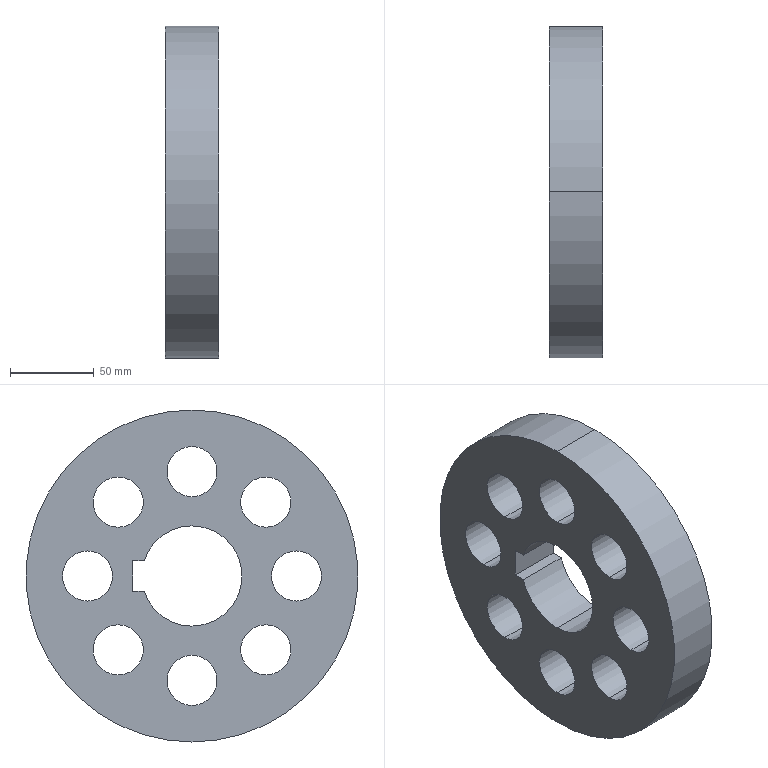Component | SolidWorks | SynchronousDrivePulley-1 | 1 solid | 26 faces | box 32 x 198.68 x 198.68 mm | volume 717277 mm3 | cylinder 21 | plane 5 | commonest cylinder face diameters 30 x16 60 x3 198.68 x2
build123d program:
from build123d import *

# Parameters (mm, degrees)
SKETCH1_R           = 99.34
SKETCH1_R_2         = 15
BOSS_EXTRUDE1_DEPTH = 16


with BuildPart() as part:
    # Sketch1 → Boss-Extrude1 (new, symmetric)
    with BuildSketch(Plane(origin=(0, 0, 0), x_dir=(0, 0, -1), z_dir=(1, 0, 0))):
        Circle(SKETCH1_R)
        with Locations((0, 62.5)):
            Circle(SKETCH1_R_2, mode=Mode.SUBTRACT)
        with Locations((44.194, 44.194)):
            Circle(SKETCH1_R_2, mode=Mode.SUBTRACT)
        with Locations((62.5, 0)):
            Circle(SKETCH1_R_2, mode=Mode.SUBTRACT)
        with Locations((44.194, -44.194)):
            Circle(SKETCH1_R_2, mode=Mode.SUBTRACT)
        with Locations((0, -62.5)):
            Circle(SKETCH1_R_2, mode=Mode.SUBTRACT)
        with Locations((-44.194, -44.194)):
            Circle(SKETCH1_R_2, mode=Mode.SUBTRACT)
        with Locations((-62.5, 0)):
            Circle(SKETCH1_R_2, mode=Mode.SUBTRACT)
        with Locations((-44.194, 44.194)):
            Circle(SKETCH1_R_2, mode=Mode.SUBTRACT)
        with BuildLine():
            Line((-9, 35.4), (9, 35.4))
            Line((9, 35.4), (9, 28.618))
            ThreePointArc((9, 28.618), (0, -30), (-9, 28.618))
            Line((-9, 28.618), (-9, 35.4))
        make_face(mode=Mode.SUBTRACT)
    extrude(amount=BOSS_EXTRUDE1_DEPTH, both=True)


solid = part.part

# Placed as in the assembly
solid = solid.moved(Location((518.553, 34.532, 0), (0, 0, 0)))
STEP:
#1=CARTESIAN_POINT('',(21.045,3.099,2.33));
#2=VERTEX_POINT('',#1);
#3=CARTESIAN_POINT('',(21.045,3.099,1.149));
#4=VERTEX_POINT('',#3);
#5=CARTESIAN_POINT('',(21.045,3.099,1.74));
#6=DIRECTION('',(1.,0.,0.));
#7=DIRECTION('',(0.,0.,-1.));
#8=AXIS2_PLACEMENT_3D('',#5,#6,#7);
#9=CIRCLE('',#8,0.5906);
#10=EDGE_CURVE('',#2,#4,#9,.T.);
#11=ORIENTED_EDGE('',*,*,#10,.T.);
#12=CARTESIAN_POINT('',(19.786,3.099,1.149));
#13=VERTEX_POINT('',#12);
#14=CARTESIAN_POINT('',(21.045,3.099,1.149));
#15=DIRECTION('',(-1.,0.,0.));
#16=VECTOR('',#15,39.37);
#17=LINE('',#14,#16);
#18=EDGE_CURVE('',#4,#13,#17,.T.);
#19=ORIENTED_EDGE('',*,*,#18,.T.);
#20=CARTESIAN_POINT('',(19.786,3.099,2.33));
#21=VERTEX_POINT('',#20);
#22=CARTESIAN_POINT('',(19.786,3.099,1.74));
#23=DIRECTION('',(1.,0.,0.));
#24=DIRECTION('',(0.,0.,-1.));
#25=AXIS2_PLACEMENT_3D('',#22,#23,#24);
#26=CIRCLE('',#25,0.5906);
#27=EDGE_CURVE('',#21,#13,#26,.T.);
#28=ORIENTED_EDGE('',*,*,#27,.F.);
#29=CARTESIAN_POINT('',(21.045,3.099,2.33));
#30=DIRECTION('',(-1.,0.,0.));
#31=VECTOR('',#30,39.37);
#32=LINE('',#29,#31);
#33=EDGE_CURVE('',#2,#21,#32,.T.);
#34=ORIENTED_EDGE('',*,*,#33,.F.);
#35=EDGE_LOOP('',(#11,#19,#28,#34));
#36=FACE_OUTER_BOUND('',#35,.T.);
#37=CARTESIAN_POINT('',(21.045,3.099,1.74));
#38=DIRECTION('',(-1.,0.,0.));
#39=DIRECTION('',(0.,0.,1.));
#40=AXIS2_PLACEMENT_3D('',#37,#38,#39);
#41=CYLINDRICAL_SURFACE('',#40,0.5906);
#42=ADVANCED_FACE('',(#36),#41,.F.);
#43=CARTESIAN_POINT('',(21.045,1.36,3.051));
#44=VERTEX_POINT('',#43);
#45=CARTESIAN_POINT('',(21.045,1.36,1.87));
#46=VERTEX_POINT('',#45);
#47=CARTESIAN_POINT('',(21.045,1.36,2.461));
#48=DIRECTION('',(1.,0.,0.));
#49=DIRECTION('',(0.,0.,-1.));
#50=AXIS2_PLACEMENT_3D('',#47,#48,#49);
#51=CIRCLE('',#50,0.5906);
#52=EDGE_CURVE('',#44,#46,#51,.T.);
#53=ORIENTED_EDGE('',*,*,#52,.T.);
#54=CARTESIAN_POINT('',(19.786,1.36,1.87));
#55=VERTEX_POINT('',#54);
#56=CARTESIAN_POINT('',(21.045,1.36,1.87));
#57=DIRECTION('',(-1.,0.,0.));
#58=VECTOR('',#57,39.37);
#59=LINE('',#56,#58);
#60=EDGE_CURVE('',#46,#55,#59,.T.);
#61=ORIENTED_EDGE('',*,*,#60,.T.);
#62=CARTESIAN_POINT('',(19.786,1.36,3.051));
#63=VERTEX_POINT('',#62);
#64=CARTESIAN_POINT('',(19.786,1.36,2.461));
#65=DIRECTION('',(1.,0.,0.));
#66=DIRECTION('',(0.,0.,-1.));
#67=AXIS2_PLACEMENT_3D('',#64,#65,#66);
#68=CIRCLE('',#67,0.5906);
#69=EDGE_CURVE('',#63,#55,#68,.T.);
#70=ORIENTED_EDGE('',*,*,#69,.F.);
#71=CARTESIAN_POINT('',(21.045,1.36,3.051));
#72=DIRECTION('',(-1.,0.,0.));
#73=VECTOR('',#72,39.37);
#74=LINE('',#71,#73);
#75=EDGE_CURVE('',#44,#63,#74,.T.);
#76=ORIENTED_EDGE('',*,*,#75,.F.);
#77=EDGE_LOOP('',(#53,#61,#70,#76));
#78=FACE_OUTER_BOUND('',#77,.T.);
#79=CARTESIAN_POINT('',(21.045,1.36,2.461));
#80=DIRECTION('',(-1.,0.,0.));
#81=DIRECTION('',(0.,0.,1.));
#82=AXIS2_PLACEMENT_3D('',#79,#80,#81);
#83=CYLINDRICAL_SURFACE('',#82,0.5906);
#84=ADVANCED_FACE('',(#78),#83,.F.);
#85=CARTESIAN_POINT('',(21.045,-0.3804,2.33));
#86=VERTEX_POINT('',#85);
#87=CARTESIAN_POINT('',(21.045,-0.3804,1.149));
#88=VERTEX_POINT('',#87);
#89=CARTESIAN_POINT('',(21.045,-0.3804,1.74));
#90=DIRECTION('',(1.,0.,0.));
#91=DIRECTION('',(0.,0.,-1.));
#92=AXIS2_PLACEMENT_3D('',#89,#90,#91);
#93=CIRCLE('',#92,0.5906);
#94=EDGE_CURVE('',#86,#88,#93,.T.);
#95=ORIENTED_EDGE('',*,*,#94,.T.);
#96=CARTESIAN_POINT('',(19.786,-0.3804,1.149));
#97=VERTEX_POINT('',#96);
#98=CARTESIAN_POINT('',(21.045,-0.3804,1.149));
#99=DIRECTION('',(-1.,0.,0.));
#100=VECTOR('',#99,39.37);
#101=LINE('',#98,#100);
#102=EDGE_CURVE('',#88,#97,#101,.T.);
#103=ORIENTED_EDGE('',*,*,#102,.T.);
#104=CARTESIAN_POINT('',(19.786,-0.3804,2.33));
#105=VERTEX_POINT('',#104);
#106=CARTESIAN_POINT('',(19.786,-0.3804,1.74));
#107=DIRECTION('',(1.,0.,0.));
#108=DIRECTION('',(0.,0.,-1.));
#109=AXIS2_PLACEMENT_3D('',#106,#107,#108);
#110=CIRCLE('',#109,0.5906);
#111=EDGE_CURVE('',#105,#97,#110,.T.);
#112=ORIENTED_EDGE('',*,*,#111,.F.);
#113=CARTESIAN_POINT('',(21.045,-0.3804,2.33));
#114=DIRECTION('',(-1.,0.,0.));
#115=VECTOR('',#114,39.37);
#116=LINE('',#113,#115);
#117=EDGE_CURVE('',#86,#105,#116,.T.);
#118=ORIENTED_EDGE('',*,*,#117,.F.);
#119=EDGE_LOOP('',(#95,#103,#112,#118));
#120=FACE_OUTER_BOUND('',#119,.T.);
#121=CARTESIAN_POINT('',(21.045,-0.3804,1.74));
#122=DIRECTION('',(-1.,0.,0.));
#123=DIRECTION('',(0.,0.,1.));
#124=AXIS2_PLACEMENT_3D('',#121,#122,#123);
#125=CYLINDRICAL_SURFACE('',#124,0.5906);
#126=ADVANCED_FACE('',(#120),#125,.F.);
#127=CARTESIAN_POINT('',(21.045,-1.101,0.5906));
#128=VERTEX_POINT('',#127);
#129=CARTESIAN_POINT('',(21.045,-1.101,-0.5906));
#130=VERTEX_POINT('',#129);
#131=CARTESIAN_POINT('',(21.045,-1.101,-0.));
#132=DIRECTION('',(1.,0.,0.));
#133=DIRECTION('',(0.,0.,-1.));
#134=AXIS2_PLACEMENT_3D('',#131,#132,#133);
#135=CIRCLE('',#134,0.5906);
#136=EDGE_CURVE('',#128,#130,#135,.T.);
#137=ORIENTED_EDGE('',*,*,#136,.T.);
#138=CARTESIAN_POINT('',(19.786,-1.101,-0.5906));
#139=VERTEX_POINT('',#138);
#140=CARTESIAN_POINT('',(21.045,-1.101,-0.5906));
#141=DIRECTION('',(-1.,0.,0.));
#142=VECTOR('',#141,39.37);
#143=LINE('',#140,#142);
#144=EDGE_CURVE('',#130,#139,#143,.T.);
#145=ORIENTED_EDGE('',*,*,#144,.T.);
#146=CARTESIAN_POINT('',(19.786,-1.101,0.5906));
#147=VERTEX_POINT('',#146);
#148=CARTESIAN_POINT('',(19.786,-1.101,-0.));
#149=DIRECTION('',(1.,0.,0.));
#150=DIRECTION('',(0.,0.,-1.));
#151=AXIS2_PLACEMENT_3D('',#148,#149,#150);
#152=CIRCLE('',#151,0.5906);
#153=EDGE_CURVE('',#147,#139,#152,.T.);
#154=ORIENTED_EDGE('',*,*,#153,.F.);
#155=CARTESIAN_POINT('',(21.045,-1.101,0.5906));
#156=DIRECTION('',(-1.,0.,0.));
#157=VECTOR('',#156,39.37);
#158=LINE('',#155,#157);
#159=EDGE_CURVE('',#128,#147,#158,.T.);
#160=ORIENTED_EDGE('',*,*,#159,.F.);
#161=EDGE_LOOP('',(#137,#145,#154,#160));
#162=FACE_OUTER_BOUND('',#161,.T.);
#163=CARTESIAN_POINT('',(21.045,-1.101,-0.));
#164=DIRECTION('',(-1.,0.,0.));
#165=DIRECTION('',(0.,0.,1.));
#166=AXIS2_PLACEMENT_3D('',#163,#164,#165);
#167=CYLINDRICAL_SURFACE('',#166,0.5906);
#168=ADVANCED_FACE('',(#162),#167,.F.);
#169=CARTESIAN_POINT('',(21.045,-0.3804,-1.149));
#170=VERTEX_POINT('',#169);
#171=CARTESIAN_POINT('',(21.045,-0.3804,-2.33));
#172=VERTEX_POINT('',#171);
#173=CARTESIAN_POINT('',(21.045,-0.3804,-1.74));
#174=DIRECTION('',(1.,0.,0.));
#175=DIRECTION('',(0.,0.,-1.));
#176=AXIS2_PLACEMENT_3D('',#173,#174,#175);
#177=CIRCLE('',#176,0.5906);
#178=EDGE_CURVE('',#170,#172,#177,.T.);
#179=ORIENTED_EDGE('',*,*,#178,.T.);
#180=CARTESIAN_POINT('',(19.786,-0.3804,-2.33));
#181=VERTEX_POINT('',#180);
#182=CARTESIAN_POINT('',(21.045,-0.3804,-2.33));
#183=DIRECTION('',(-1.,0.,0.));
#184=VECTOR('',#183,39.37);
#185=LINE('',#182,#184);
#186=EDGE_CURVE('',#172,#181,#185,.T.);
#187=ORIENTED_EDGE('',*,*,#186,.T.);
#188=CARTESIAN_POINT('',(19.786,-0.3804,-1.149));
#189=VERTEX_POINT('',#188);
#190=CARTESIAN_POINT('',(19.786,-0.3804,-1.74));
#191=DIRECTION('',(1.,0.,0.));
#192=DIRECTION('',(0.,0.,-1.));
#193=AXIS2_PLACEMENT_3D('',#190,#191,#192);
#194=CIRCLE('',#193,0.5906);
#195=EDGE_CURVE('',#189,#181,#194,.T.);
#196=ORIENTED_EDGE('',*,*,#195,.F.);
#197=CARTESIAN_POINT('',(21.045,-0.3804,-1.149));
#198=DIRECTION('',(-1.,0.,0.));
#199=VECTOR('',#198,39.37);
#200=LINE('',#197,#199);
#201=EDGE_CURVE('',#170,#189,#200,.T.);
#202=ORIENTED_EDGE('',*,*,#201,.F.);
#203=EDGE_LOOP('',(#179,#187,#196,#202));
#204=FACE_OUTER_BOUND('',#203,.T.);
#205=CARTESIAN_POINT('',(21.045,-0.3804,-1.74));
#206=DIRECTION('',(-1.,0.,0.));
#207=DIRECTION('',(0.,0.,1.));
#208=AXIS2_PLACEMENT_3D('',#205,#206,#207);
#209=CYLINDRICAL_SURFACE('',#208,0.5906);
#210=ADVANCED_FACE('',(#204),#209,.F.);
#211=CARTESIAN_POINT('',(21.045,1.36,-1.87));
#212=VERTEX_POINT('',#211);
#213=CARTESIAN_POINT('',(21.045,1.36,-3.051));
#214=VERTEX_POINT('',#213);
#215=CARTESIAN_POINT('',(21.045,1.36,-2.461));
#216=DIRECTION('',(1.,0.,0.));
#217=DIRECTION('',(0.,0.,-1.));
#218=AXIS2_PLACEMENT_3D('',#215,#216,#217);
#219=CIRCLE('',#218,0.5906);
#220=EDGE_CURVE('',#212,#214,#219,.T.);
#221=ORIENTED_EDGE('',*,*,#220,.T.);
#222=CARTESIAN_POINT('',(19.786,1.36,-3.051));
#223=VERTEX_POINT('',#222);
#224=CARTESIAN_POINT('',(21.045,1.36,-3.051));
#225=DIRECTION('',(-1.,0.,0.));
#226=VECTOR('',#225,39.37);
#227=LINE('',#224,#226);
#228=EDGE_CURVE('',#214,#223,#227,.T.);
#229=ORIENTED_EDGE('',*,*,#228,.T.);
#230=CARTESIAN_POINT('',(19.786,1.36,-1.87));
#231=VERTEX_POINT('',#230);
#232=CARTESIAN_POINT('',(19.786,1.36,-2.461));
#233=DIRECTION('',(1.,0.,0.));
#234=DIRECTION('',(0.,0.,-1.));
#235=AXIS2_PLACEMENT_3D('',#232,#233,#234);
#236=CIRCLE('',#235,0.5906);
#237=EDGE_CURVE('',#231,#223,#236,.T.);
#238=ORIENTED_EDGE('',*,*,#237,.F.);
#239=CARTESIAN_POINT('',(21.045,1.36,-1.87));
#240=DIRECTION('',(-1.,0.,0.));
#241=VECTOR('',#240,39.37);
#242=LINE('',#239,#241);
#243=EDGE_CURVE('',#212,#231,#242,.T.);
#244=ORIENTED_EDGE('',*,*,#243,.F.);
#245=EDGE_LOOP('',(#221,#229,#238,#244));
#246=FACE_OUTER_BOUND('',#245,.T.);
#247=CARTESIAN_POINT('',(21.045,1.36,-2.461));
#248=DIRECTION('',(-1.,0.,0.));
#249=DIRECTION('',(0.,0.,1.));
#250=AXIS2_PLACEMENT_3D('',#247,#248,#249);
#251=CYLINDRICAL_SURFACE('',#250,0.5906);
#252=ADVANCED_FACE('',(#246),#251,.F.);
#253=CARTESIAN_POINT('',(21.045,3.099,-1.149));
#254=VERTEX_POINT('',#253);
#255=CARTESIAN_POINT('',(21.045,3.099,-2.33));
#256=VERTEX_POINT('',#255);
#257=CARTESIAN_POINT('',(21.045,3.099,-1.74));
#258=DIRECTION('',(1.,0.,0.));
#259=DIRECTION('',(0.,0.,-1.));
#260=AXIS2_PLACEMENT_3D('',#257,#258,#259);
#261=CIRCLE('',#260,0.5906);
#262=EDGE_CURVE('',#254,#256,#261,.T.);
#263=ORIENTED_EDGE('',*,*,#262,.T.);
#264=CARTESIAN_POINT('',(19.786,3.099,-2.33));
#265=VERTEX_POINT('',#264);
#266=CARTESIAN_POINT('',(21.045,3.099,-2.33));
#267=DIRECTION('',(-1.,0.,0.));
#268=VECTOR('',#267,39.37);
#269=LINE('',#266,#268);
#270=EDGE_CURVE('',#256,#265,#269,.T.);
#271=ORIENTED_EDGE('',*,*,#270,.T.);
#272=CARTESIAN_POINT('',(19.786,3.099,-1.149));
#273=VERTEX_POINT('',#272);
#274=CARTESIAN_POINT('',(19.786,3.099,-1.74));
#275=DIRECTION('',(1.,0.,0.));
#276=DIRECTION('',(0.,0.,-1.));
#277=AXIS2_PLACEMENT_3D('',#274,#275,#276);
#278=CIRCLE('',#277,0.5906);
#279=EDGE_CURVE('',#273,#265,#278,.T.);
#280=ORIENTED_EDGE('',*,*,#279,.F.);
#281=CARTESIAN_POINT('',(21.045,3.099,-1.149));
#282=DIRECTION('',(-1.,0.,0.));
#283=VECTOR('',#282,39.37);
#284=LINE('',#281,#283);
#285=EDGE_CURVE('',#254,#273,#284,.T.);
#286=ORIENTED_EDGE('',*,*,#285,.F.);
#287=EDGE_LOOP('',(#263,#271,#280,#286));
#288=FACE_OUTER_BOUND('',#287,.T.);
#289=CARTESIAN_POINT('',(21.045,3.099,-1.74));
#290=DIRECTION('',(-1.,0.,0.));
#291=DIRECTION('',(0.,0.,1.));
#292=AXIS2_PLACEMENT_3D('',#289,#290,#291);
#293=CYLINDRICAL_SURFACE('',#292,0.5906);
#294=ADVANCED_FACE('',(#288),#293,.F.);
#295=CARTESIAN_POINT('',(21.045,3.82,0.5906));
#296=VERTEX_POINT('',#295);
#297=CARTESIAN_POINT('',(21.045,3.82,-0.5906));
#298=VERTEX_POINT('',#297);
#299=CARTESIAN_POINT('',(21.045,3.82,0.));
#300=DIRECTION('',(1.,0.,0.));
#301=DIRECTION('',(0.,0.,-1.));
#302=AXIS2_PLACEMENT_3D('',#299,#300,#301);
#303=CIRCLE('',#302,0.5906);
#304=EDGE_CURVE('',#296,#298,#303,.T.);
#305=ORIENTED_EDGE('',*,*,#304,.T.);
#306=CARTESIAN_POINT('',(19.786,3.82,-0.5906));
#307=VERTEX_POINT('',#306);
#308=CARTESIAN_POINT('',(21.045,3.82,-0.5906));
#309=DIRECTION('',(-1.,0.,0.));
#310=VECTOR('',#309,39.37);
#311=LINE('',#308,#310);
#312=EDGE_CURVE('',#298,#307,#311,.T.);
#313=ORIENTED_EDGE('',*,*,#312,.T.);
#314=CARTESIAN_POINT('',(19.786,3.82,0.5906));
#315=VERTEX_POINT('',#314);
#316=CARTESIAN_POINT('',(19.786,3.82,0.));
#317=DIRECTION('',(1.,0.,0.));
#318=DIRECTION('',(0.,0.,-1.));
#319=AXIS2_PLACEMENT_3D('',#316,#317,#318);
#320=CIRCLE('',#319,0.5906);
#321=EDGE_CURVE('',#315,#307,#320,.T.);
#322=ORIENTED_EDGE('',*,*,#321,.F.);
#323=CARTESIAN_POINT('',(21.045,3.82,0.5906));
#324=DIRECTION('',(-1.,0.,0.));
#325=VECTOR('',#324,39.37);
#326=LINE('',#323,#325);
#327=EDGE_CURVE('',#296,#315,#326,.T.);
#328=ORIENTED_EDGE('',*,*,#327,.F.);
#329=EDGE_LOOP('',(#305,#313,#322,#328));
#330=FACE_OUTER_BOUND('',#329,.T.);
#331=CARTESIAN_POINT('',(21.045,3.82,0.));
#332=DIRECTION('',(-1.,0.,0.));
#333=DIRECTION('',(0.,0.,1.));
#334=AXIS2_PLACEMENT_3D('',#331,#332,#333);
#335=CYLINDRICAL_SURFACE('',#334,0.5906);
#336=ADVANCED_FACE('',(#330),#335,.F.);
#337=CARTESIAN_POINT('',(21.045,1.36,1.181));
#338=VERTEX_POINT('',#337);
#339=CARTESIAN_POINT('',(21.045,1.36,-1.181));
#340=VERTEX_POINT('',#339);
#341=CARTESIAN_POINT('',(21.045,1.36,0.));
#342=DIRECTION('',(1.,0.,0.));
#343=DIRECTION('',(0.,0.,-1.));
#344=AXIS2_PLACEMENT_3D('',#341,#342,#343);
#345=CIRCLE('',#344,1.181);
#346=EDGE_CURVE('',#338,#340,#345,.T.);
#347=ORIENTED_EDGE('',*,*,#346,.T.);
#348=CARTESIAN_POINT('',(19.786,1.36,-1.181));
#349=VERTEX_POINT('',#348);
#350=CARTESIAN_POINT('',(21.045,1.36,-1.181));
#351=DIRECTION('',(-1.,0.,0.));
#352=VECTOR('',#351,39.37);
#353=LINE('',#350,#352);
#354=EDGE_CURVE('',#340,#349,#353,.T.);
#355=ORIENTED_EDGE('',*,*,#354,.T.);
#356=CARTESIAN_POINT('',(19.786,1.36,1.181));
#357=VERTEX_POINT('',#356);
#358=CARTESIAN_POINT('',(19.786,1.36,0.));
#359=DIRECTION('',(1.,0.,0.));
#360=DIRECTION('',(0.,0.,-1.));
#361=AXIS2_PLACEMENT_3D('',#358,#359,#360);
#362=CIRCLE('',#361,1.181);
#363=EDGE_CURVE('',#357,#349,#362,.T.);
#364=ORIENTED_EDGE('',*,*,#363,.F.);
#365=CARTESIAN_POINT('',(21.045,1.36,1.181));
#366=DIRECTION('',(-1.,0.,0.));
#367=VECTOR('',#366,39.37);
#368=LINE('',#365,#367);
#369=EDGE_CURVE('',#338,#357,#368,.T.);
#370=ORIENTED_EDGE('',*,*,#369,.F.);
#371=EDGE_LOOP('',(#347,#355,#364,#370));
#372=FACE_OUTER_BOUND('',#371,.T.);
#373=CARTESIAN_POINT('',(21.045,1.36,0.));
#374=DIRECTION('',(-1.,0.,0.));
#375=DIRECTION('',(0.,0.,1.));
#376=AXIS2_PLACEMENT_3D('',#373,#374,#375);
#377=CYLINDRICAL_SURFACE('',#376,1.181);
#378=ADVANCED_FACE('',(#372),#377,.F.);
#379=CARTESIAN_POINT('',(21.045,2.486,0.3543));
#380=VERTEX_POINT('',#379);
#381=CARTESIAN_POINT('',(21.045,1.36,0.));
#382=DIRECTION('',(1.,0.,0.));
#383=DIRECTION('',(0.,0.,-1.));
#384=AXIS2_PLACEMENT_3D('',#381,#382,#383);
#385=CIRCLE('',#384,1.181);
#386=EDGE_CURVE('',#380,#338,#385,.T.);
#387=ORIENTED_EDGE('',*,*,#386,.T.);
#388=ORIENTED_EDGE('',*,*,#369,.T.);
#389=CARTESIAN_POINT('',(19.786,2.486,0.3543));
#390=VERTEX_POINT('',#389);
#391=CARTESIAN_POINT('',(19.786,1.36,0.));
#392=DIRECTION('',(1.,0.,0.));
#393=DIRECTION('',(0.,0.,-1.));
#394=AXIS2_PLACEMENT_3D('',#391,#392,#393);
#395=CIRCLE('',#394,1.181);
#396=EDGE_CURVE('',#390,#357,#395,.T.);
#397=ORIENTED_EDGE('',*,*,#396,.F.);
#398=CARTESIAN_POINT('',(21.045,2.486,0.3543));
#399=DIRECTION('',(-1.,0.,0.));
#400=VECTOR('',#399,39.37);
#401=LINE('',#398,#400);
#402=EDGE_CURVE('',#380,#390,#401,.T.);
#403=ORIENTED_EDGE('',*,*,#402,.F.);
#404=EDGE_LOOP('',(#387,#388,#397,#403));
#405=FACE_OUTER_BOUND('',#404,.T.);
#406=CARTESIAN_POINT('',(21.045,1.36,0.));
#407=DIRECTION('',(-1.,0.,0.));
#408=DIRECTION('',(0.,0.,1.));
#409=AXIS2_PLACEMENT_3D('',#406,#407,#408);
#410=CYLINDRICAL_SURFACE('',#409,1.181);
#411=ADVANCED_FACE('',(#405),#410,.F.);
#412=CARTESIAN_POINT('',(21.045,1.36,-3.911));
#413=VERTEX_POINT('',#412);
#414=CARTESIAN_POINT('',(21.045,1.36,3.911));
#415=VERTEX_POINT('',#414);
#416=CARTESIAN_POINT('',(21.045,1.36,0.));
#417=DIRECTION('',(1.,0.,0.));
#418=DIRECTION('',(0.,0.,-1.));
#419=AXIS2_PLACEMENT_3D('',#416,#417,#418);
#420=CIRCLE('',#419,3.911);
#421=EDGE_CURVE('',#413,#415,#420,.T.);
#422=ORIENTED_EDGE('',*,*,#421,.F.);
#423=CARTESIAN_POINT('',(19.786,1.36,-3.911));
#424=VERTEX_POINT('',#423);
#425=CARTESIAN_POINT('',(21.045,1.36,-3.911));
#426=DIRECTION('',(-1.,0.,0.));
#427=VECTOR('',#426,39.37);
#428=LINE('',#425,#427);
#429=EDGE_CURVE('',#413,#424,#428,.T.);
#430=ORIENTED_EDGE('',*,*,#429,.T.);
#431=CARTESIAN_POINT('',(19.786,1.36,3.911));
#432=VERTEX_POINT('',#431);
#433=CARTESIAN_POINT('',(19.786,1.36,0.));
#434=DIRECTION('',(1.,0.,0.));
#435=DIRECTION('',(0.,0.,-1.));
#436=AXIS2_PLACEMENT_3D('',#433,#434,#435);
#437=CIRCLE('',#436,3.911);
#438=EDGE_CURVE('',#424,#432,#437,.T.);
#439=ORIENTED_EDGE('',*,*,#438,.T.);
#440=CARTESIAN_POINT('',(21.045,1.36,3.911));
#441=DIRECTION('',(-1.,0.,0.));
#442=VECTOR('',#441,39.37);
#443=LINE('',#440,#442);
#444=EDGE_CURVE('',#415,#432,#443,.T.);
#445=ORIENTED_EDGE('',*,*,#444,.F.);
#446=EDGE_LOOP('',(#422,#430,#439,#445));
#447=FACE_OUTER_BOUND('',#446,.T.);
#448=CARTESIAN_POINT('',(21.045,1.36,0.));
#449=DIRECTION('',(-1.,0.,0.));
#450=DIRECTION('',(0.,0.,1.));
#451=AXIS2_PLACEMENT_3D('',#448,#449,#450);
#452=CYLINDRICAL_SURFACE('',#451,3.911);
#453=ADVANCED_FACE('',(#447),#452,.T.);
#454=ORIENTED_EDGE('',*,*,#52,.F.);
#455=CARTESIAN_POINT('',(21.045,1.36,2.461));
#456=DIRECTION('',(1.,0.,0.));
#457=DIRECTION('',(0.,0.,-1.));
#458=AXIS2_PLACEMENT_3D('',#455,#456,#457);
#459=CIRCLE('',#458,0.5906);
#460=EDGE_CURVE('',#46,#44,#459,.T.);
#461=ORIENTED_EDGE('',*,*,#460,.F.);
#462=EDGE_LOOP('',(#454,#461));
#463=FACE_BOUND('',#462,.T.);
#464=ORIENTED_EDGE('',*,*,#136,.F.);
#465=CARTESIAN_POINT('',(21.045,-1.101,-0.));
#466=DIRECTION('',(1.,0.,0.));
#467=DIRECTION('',(0.,0.,-1.));
#468=AXIS2_PLACEMENT_3D('',#465,#466,#467);
#469=CIRCLE('',#468,0.5906);
#470=EDGE_CURVE('',#130,#128,#469,.T.);
#471=ORIENTED_EDGE('',*,*,#470,.F.);
#472=EDGE_LOOP('',(#464,#471));
#473=FACE_BOUND('',#472,.T.);
#474=ORIENTED_EDGE('',*,*,#220,.F.);
#475=CARTESIAN_POINT('',(21.045,1.36,-2.461));
#476=DIRECTION('',(1.,0.,0.));
#477=DIRECTION('',(0.,0.,-1.));
#478=AXIS2_PLACEMENT_3D('',#475,#476,#477);
#479=CIRCLE('',#478,0.5906);
#480=EDGE_CURVE('',#214,#212,#479,.T.);
#481=ORIENTED_EDGE('',*,*,#480,.F.);
#482=EDGE_LOOP('',(#474,#481));
#483=FACE_BOUND('',#482,.T.);
#484=ORIENTED_EDGE('',*,*,#304,.F.);
#485=CARTESIAN_POINT('',(21.045,3.82,0.));
#486=DIRECTION('',(1.,0.,0.));
#487=DIRECTION('',(0.,0.,-1.));
#488=AXIS2_PLACEMENT_3D('',#485,#486,#487);
#489=CIRCLE('',#488,0.5906);
#490=EDGE_CURVE('',#298,#296,#489,.T.);
#491=ORIENTED_EDGE('',*,*,#490,.F.);
#492=EDGE_LOOP('',(#484,#491));
#493=FACE_BOUND('',#492,.T.);
#494=CARTESIAN_POINT('',(21.045,1.36,0.));
#495=DIRECTION('',(1.,0.,0.));
#496=DIRECTION('',(0.,0.,-1.));
#497=AXIS2_PLACEMENT_3D('',#494,#495,#496);
#498=CIRCLE('',#497,3.911);
#499=EDGE_CURVE('',#415,#413,#498,.T.);
#500=ORIENTED_EDGE('',*,*,#499,.T.);
#501=ORIENTED_EDGE('',*,*,#421,.T.);
#502=EDGE_LOOP('',(#500,#501));
#503=FACE_OUTER_BOUND('',#502,.T.);
#504=ORIENTED_EDGE('',*,*,#386,.F.);
#505=CARTESIAN_POINT('',(21.045,2.753,0.3543));
#506=VERTEX_POINT('',#505);
#507=CARTESIAN_POINT('',(21.045,2.753,0.3543));
#508=DIRECTION('',(0.,-1.,0.));
#509=VECTOR('',#508,39.37);
#510=LINE('',#507,#509);
#511=EDGE_CURVE('',#506,#380,#510,.T.);
#512=ORIENTED_EDGE('',*,*,#511,.F.);
#513=CARTESIAN_POINT('',(21.045,2.753,-0.3543));
#514=VERTEX_POINT('',#513);
#515=CARTESIAN_POINT('',(21.045,2.753,0.3543));
#516=DIRECTION('',(0.,0.,1.));
#517=VECTOR('',#516,39.37);
#518=LINE('',#515,#517);
#519=EDGE_CURVE('',#514,#506,#518,.T.);
#520=ORIENTED_EDGE('',*,*,#519,.F.);
#521=CARTESIAN_POINT('',(21.045,2.486,-0.3543));
#522=VERTEX_POINT('',#521);
#523=CARTESIAN_POINT('',(21.045,2.753,-0.3543));
#524=DIRECTION('',(0.,1.,0.));
#525=VECTOR('',#524,39.37);
#526=LINE('',#523,#525);
#527=EDGE_CURVE('',#522,#514,#526,.T.);
#528=ORIENTED_EDGE('',*,*,#527,.F.);
#529=CARTESIAN_POINT('',(21.045,1.36,0.));
#530=DIRECTION('',(1.,0.,0.));
#531=DIRECTION('',(0.,0.,-1.));
#532=AXIS2_PLACEMENT_3D('',#529,#530,#531);
#533=CIRCLE('',#532,1.181);
#534=EDGE_CURVE('',#340,#522,#533,.T.);
#535=ORIENTED_EDGE('',*,*,#534,.F.);
#536=ORIENTED_EDGE('',*,*,#346,.F.);
#537=EDGE_LOOP('',(#504,#512,#520,#528,#535,#536));
#538=FACE_BOUND('',#537,.T.);
#539=ORIENTED_EDGE('',*,*,#262,.F.);
#540=CARTESIAN_POINT('',(21.045,3.099,-1.74));
#541=DIRECTION('',(1.,0.,0.));
#542=DIRECTION('',(0.,0.,-1.));
#543=AXIS2_PLACEMENT_3D('',#540,#541,#542);
#544=CIRCLE('',#543,0.5906);
#545=EDGE_CURVE('',#256,#254,#544,.T.);
#546=ORIENTED_EDGE('',*,*,#545,.F.);
#547=EDGE_LOOP('',(#539,#546));
#548=FACE_BOUND('',#547,.T.);
#549=ORIENTED_EDGE('',*,*,#178,.F.);
#550=CARTESIAN_POINT('',(21.045,-0.3804,-1.74));
#551=DIRECTION('',(1.,0.,0.));
#552=DIRECTION('',(0.,0.,-1.));
#553=AXIS2_PLACEMENT_3D('',#550,#551,#552);
#554=CIRCLE('',#553,0.5906);
#555=EDGE_CURVE('',#172,#170,#554,.T.);
#556=ORIENTED_EDGE('',*,*,#555,.F.);
#557=EDGE_LOOP('',(#549,#556));
#558=FACE_BOUND('',#557,.T.);
#559=ORIENTED_EDGE('',*,*,#94,.F.);
#560=CARTESIAN_POINT('',(21.045,-0.3804,1.74));
#561=DIRECTION('',(1.,0.,0.));
#562=DIRECTION('',(0.,0.,-1.));
#563=AXIS2_PLACEMENT_3D('',#560,#561,#562);
#564=CIRCLE('',#563,0.5906);
#565=EDGE_CURVE('',#88,#86,#564,.T.);
#566=ORIENTED_EDGE('',*,*,#565,.F.);
#567=EDGE_LOOP('',(#559,#566));
#568=FACE_BOUND('',#567,.T.);
#569=ORIENTED_EDGE('',*,*,#10,.F.);
#570=CARTESIAN_POINT('',(21.045,3.099,1.74));
#571=DIRECTION('',(1.,0.,0.));
#572=DIRECTION('',(0.,0.,-1.));
#573=AXIS2_PLACEMENT_3D('',#570,#571,#572);
#574=CIRCLE('',#573,0.5906);
#575=EDGE_CURVE('',#4,#2,#574,.T.);
#576=ORIENTED_EDGE('',*,*,#575,.F.);
#577=EDGE_LOOP('',(#569,#576));
#578=FACE_BOUND('',#577,.T.);
#579=CARTESIAN_POINT('',(21.045,1.36,0.));
#580=DIRECTION('',(1.,0.,0.));
#581=DIRECTION('',(0.,0.,-1.));
#582=AXIS2_PLACEMENT_3D('',#579,#580,#581);
#583=PLANE('',#582);
#584=ADVANCED_FACE('',(#463,#473,#483,#493,#503,#538,#548,#558,#568,#578),#583,.T.);
#585=ORIENTED_EDGE('',*,*,#69,.T.);
#586=CARTESIAN_POINT('',(19.786,1.36,2.461));
#587=DIRECTION('',(1.,0.,0.));
#588=DIRECTION('',(0.,0.,-1.));
#589=AXIS2_PLACEMENT_3D('',#586,#587,#588);
#590=CIRCLE('',#589,0.5906);
#591=EDGE_CURVE('',#55,#63,#590,.T.);
#592=ORIENTED_EDGE('',*,*,#591,.T.);
#593=EDGE_LOOP('',(#585,#592));
#594=FACE_BOUND('',#593,.T.);
#595=ORIENTED_EDGE('',*,*,#153,.T.);
#596=CARTESIAN_POINT('',(19.786,-1.101,-0.));
#597=DIRECTION('',(1.,0.,0.));
#598=DIRECTION('',(0.,0.,-1.));
#599=AXIS2_PLACEMENT_3D('',#596,#597,#598);
#600=CIRCLE('',#599,0.5906);
#601=EDGE_CURVE('',#139,#147,#600,.T.);
#602=ORIENTED_EDGE('',*,*,#601,.T.);
#603=EDGE_LOOP('',(#595,#602));
#604=FACE_BOUND('',#603,.T.);
#605=ORIENTED_EDGE('',*,*,#237,.T.);
#606=CARTESIAN_POINT('',(19.786,1.36,-2.461));
#607=DIRECTION('',(1.,0.,0.));
#608=DIRECTION('',(0.,0.,-1.));
#609=AXIS2_PLACEMENT_3D('',#606,#607,#608);
#610=CIRCLE('',#609,0.5906);
#611=EDGE_CURVE('',#223,#231,#610,.T.);
#612=ORIENTED_EDGE('',*,*,#611,.T.);
#613=EDGE_LOOP('',(#605,#612));
#614=FACE_BOUND('',#613,.T.);
#615=ORIENTED_EDGE('',*,*,#321,.T.);
#616=CARTESIAN_POINT('',(19.786,3.82,0.));
#617=DIRECTION('',(1.,0.,0.));
#618=DIRECTION('',(0.,0.,-1.));
#619=AXIS2_PLACEMENT_3D('',#616,#617,#618);
#620=CIRCLE('',#619,0.5906);
#621=EDGE_CURVE('',#307,#315,#620,.T.);
#622=ORIENTED_EDGE('',*,*,#621,.T.);
#623=EDGE_LOOP('',(#615,#622));
#624=FACE_BOUND('',#623,.T.);
#625=CARTESIAN_POINT('',(19.786,1.36,0.));
#626=DIRECTION('',(1.,0.,0.));
#627=DIRECTION('',(0.,0.,-1.));
#628=AXIS2_PLACEMENT_3D('',#625,#626,#627);
#629=CIRCLE('',#628,3.911);
#630=EDGE_CURVE('',#432,#424,#629,.T.);
#631=ORIENTED_EDGE('',*,*,#630,.F.);
#632=ORIENTED_EDGE('',*,*,#438,.F.);
#633=EDGE_LOOP('',(#631,#632));
#634=FACE_OUTER_BOUND('',#633,.T.);
#635=CARTESIAN_POINT('',(19.786,2.753,0.3543));
#636=VERTEX_POINT('',#635);
#637=CARTESIAN_POINT('',(19.786,2.753,0.3543));
#638=DIRECTION('',(0.,-1.,0.));
#639=VECTOR('',#638,39.37);
#640=LINE('',#637,#639);
#641=EDGE_CURVE('',#636,#390,#640,.T.);
#642=ORIENTED_EDGE('',*,*,#641,.T.);
#643=ORIENTED_EDGE('',*,*,#396,.T.);
#644=ORIENTED_EDGE('',*,*,#363,.T.);
#645=CARTESIAN_POINT('',(19.786,2.486,-0.3543));
#646=VERTEX_POINT('',#645);
#647=CARTESIAN_POINT('',(19.786,1.36,0.));
#648=DIRECTION('',(1.,0.,0.));
#649=DIRECTION('',(0.,0.,-1.));
#650=AXIS2_PLACEMENT_3D('',#647,#648,#649);
#651=CIRCLE('',#650,1.181);
#652=EDGE_CURVE('',#349,#646,#651,.T.);
#653=ORIENTED_EDGE('',*,*,#652,.T.);
#654=CARTESIAN_POINT('',(19.786,2.753,-0.3543));
#655=VERTEX_POINT('',#654);
#656=CARTESIAN_POINT('',(19.786,2.753,-0.3543));
#657=DIRECTION('',(0.,1.,0.));
#658=VECTOR('',#657,39.37);
#659=LINE('',#656,#658);
#660=EDGE_CURVE('',#646,#655,#659,.T.);
#661=ORIENTED_EDGE('',*,*,#660,.T.);
#662=CARTESIAN_POINT('',(19.786,2.753,0.3543));
#663=DIRECTION('',(0.,0.,1.));
#664=VECTOR('',#663,39.37);
#665=LINE('',#662,#664);
#666=EDGE_CURVE('',#655,#636,#665,.T.);
#667=ORIENTED_EDGE('',*,*,#666,.T.);
#668=EDGE_LOOP('',(#642,#643,#644,#653,#661,#667));
#669=FACE_BOUND('',#668,.T.);
#670=ORIENTED_EDGE('',*,*,#279,.T.);
#671=CARTESIAN_POINT('',(19.786,3.099,-1.74));
#672=DIRECTION('',(1.,0.,0.));
#673=DIRECTION('',(0.,0.,-1.));
#674=AXIS2_PLACEMENT_3D('',#671,#672,#673);
#675=CIRCLE('',#674,0.5906);
#676=EDGE_CURVE('',#265,#273,#675,.T.);
#677=ORIENTED_EDGE('',*,*,#676,.T.);
#678=EDGE_LOOP('',(#670,#677));
#679=FACE_BOUND('',#678,.T.);
#680=ORIENTED_EDGE('',*,*,#195,.T.);
#681=CARTESIAN_POINT('',(19.786,-0.3804,-1.74));
#682=DIRECTION('',(1.,0.,0.));
#683=DIRECTION('',(0.,0.,-1.));
#684=AXIS2_PLACEMENT_3D('',#681,#682,#683);
#685=CIRCLE('',#684,0.5906);
#686=EDGE_CURVE('',#181,#189,#685,.T.);
#687=ORIENTED_EDGE('',*,*,#686,.T.);
#688=EDGE_LOOP('',(#680,#687));
#689=FACE_BOUND('',#688,.T.);
#690=ORIENTED_EDGE('',*,*,#111,.T.);
#691=CARTESIAN_POINT('',(19.786,-0.3804,1.74));
#692=DIRECTION('',(1.,0.,0.));
#693=DIRECTION('',(0.,0.,-1.));
#694=AXIS2_PLACEMENT_3D('',#691,#692,#693);
#695=CIRCLE('',#694,0.5906);
#696=EDGE_CURVE('',#97,#105,#695,.T.);
#697=ORIENTED_EDGE('',*,*,#696,.T.);
#698=EDGE_LOOP('',(#690,#697));
#699=FACE_BOUND('',#698,.T.);
#700=ORIENTED_EDGE('',*,*,#27,.T.);
#701=CARTESIAN_POINT('',(19.786,3.099,1.74));
#702=DIRECTION('',(1.,0.,0.));
#703=DIRECTION('',(0.,0.,-1.));
#704=AXIS2_PLACEMENT_3D('',#701,#702,#703);
#705=CIRCLE('',#704,0.5906);
#706=EDGE_CURVE('',#13,#21,#705,.T.);
#707=ORIENTED_EDGE('',*,*,#706,.T.);
#708=EDGE_LOOP('',(#700,#707));
#709=FACE_BOUND('',#708,.T.);
#710=CARTESIAN_POINT('',(19.786,1.36,0.));
#711=DIRECTION('',(1.,0.,0.));
#712=DIRECTION('',(0.,0.,-1.));
#713=AXIS2_PLACEMENT_3D('',#710,#711,#712);
#714=PLANE('',#713);
#715=ADVANCED_FACE('',(#594,#604,#614,#624,#634,#669,#679,#689,#699,#709),#714,.F.);
#716=ORIENTED_EDGE('',*,*,#429,.F.);
#717=ORIENTED_EDGE('',*,*,#499,.F.);
#718=ORIENTED_EDGE('',*,*,#444,.T.);
#719=ORIENTED_EDGE('',*,*,#630,.T.);
#720=EDGE_LOOP('',(#716,#717,#718,#719));
#721=FACE_OUTER_BOUND('',#720,.T.);
#722=CARTESIAN_POINT('',(21.045,1.36,0.));
#723=DIRECTION('',(-1.,0.,0.));
#724=DIRECTION('',(0.,0.,1.));
#725=AXIS2_PLACEMENT_3D('',#722,#723,#724);
#726=CYLINDRICAL_SURFACE('',#725,3.911);
#727=ADVANCED_FACE('',(#721),#726,.T.);
#728=ORIENTED_EDGE('',*,*,#641,.F.);
#729=CARTESIAN_POINT('',(21.045,2.753,0.3543));
#730=DIRECTION('',(-1.,0.,0.));
#731=VECTOR('',#730,39.37);
#732=LINE('',#729,#731);
#733=EDGE_CURVE('',#506,#636,#732,.T.);
#734=ORIENTED_EDGE('',*,*,#733,.F.);
#735=ORIENTED_EDGE('',*,*,#511,.T.);
#736=ORIENTED_EDGE('',*,*,#402,.T.);
#737=EDGE_LOOP('',(#728,#734,#735,#736));
#738=FACE_OUTER_BOUND('',#737,.T.);
#739=CARTESIAN_POINT('',(21.045,2.753,0.3543));
#740=DIRECTION('',(0.,0.,-1.));
#741=DIRECTION('',(-1.,0.,0.));
#742=AXIS2_PLACEMENT_3D('',#739,#740,#741);
#743=PLANE('',#742);
#744=ADVANCED_FACE('',(#738),#743,.T.);
#745=ORIENTED_EDGE('',*,*,#354,.F.);
#746=ORIENTED_EDGE('',*,*,#534,.T.);
#747=CARTESIAN_POINT('',(21.045,2.486,-0.3543));
#748=DIRECTION('',(-1.,0.,0.));
#749=VECTOR('',#748,39.37);
#750=LINE('',#747,#749);
#751=EDGE_CURVE('',#522,#646,#750,.T.);
#752=ORIENTED_EDGE('',*,*,#751,.T.);
#753=ORIENTED_EDGE('',*,*,#652,.F.);
#754=EDGE_LOOP('',(#745,#746,#752,#753));
#755=FACE_OUTER_BOUND('',#754,.T.);
#756=CARTESIAN_POINT('',(21.045,1.36,0.));
#757=DIRECTION('',(-1.,0.,0.));
#758=DIRECTION('',(0.,0.,1.));
#759=AXIS2_PLACEMENT_3D('',#756,#757,#758);
#760=CYLINDRICAL_SURFACE('',#759,1.181);
#761=ADVANCED_FACE('',(#755),#760,.F.);
#762=ORIENTED_EDGE('',*,*,#660,.F.);
#763=ORIENTED_EDGE('',*,*,#751,.F.);
#764=ORIENTED_EDGE('',*,*,#527,.T.);
#765=CARTESIAN_POINT('',(21.045,2.753,-0.3543));
#766=DIRECTION('',(-1.,0.,0.));
#767=VECTOR('',#766,39.37);
#768=LINE('',#765,#767);
#769=EDGE_CURVE('',#514,#655,#768,.T.);
#770=ORIENTED_EDGE('',*,*,#769,.T.);
#771=EDGE_LOOP('',(#762,#763,#764,#770));
#772=FACE_OUTER_BOUND('',#771,.T.);
#773=CARTESIAN_POINT('',(21.045,2.753,-0.3543));
#774=DIRECTION('',(0.,-0.,1.));
#775=DIRECTION('',(0.,-1.,-0.));
#776=AXIS2_PLACEMENT_3D('',#773,#774,#775);
#777=PLANE('',#776);
#778=ADVANCED_FACE('',(#772),#777,.T.);
#779=ORIENTED_EDGE('',*,*,#666,.F.);
#780=ORIENTED_EDGE('',*,*,#769,.F.);
#781=ORIENTED_EDGE('',*,*,#519,.T.);
#782=ORIENTED_EDGE('',*,*,#733,.T.);
#783=EDGE_LOOP('',(#779,#780,#781,#782));
#784=FACE_OUTER_BOUND('',#783,.T.);
#785=CARTESIAN_POINT('',(21.045,2.753,0.3543));
#786=DIRECTION('',(0.,-1.,0.));
#787=DIRECTION('',(0.,0.,-1.));
#788=AXIS2_PLACEMENT_3D('',#785,#786,#787);
#789=PLANE('',#788);
#790=ADVANCED_FACE('',(#784),#789,.T.);
#791=ORIENTED_EDGE('',*,*,#312,.F.);
#792=ORIENTED_EDGE('',*,*,#490,.T.);
#793=ORIENTED_EDGE('',*,*,#327,.T.);
#794=ORIENTED_EDGE('',*,*,#621,.F.);
#795=EDGE_LOOP('',(#791,#792,#793,#794));
#796=FACE_OUTER_BOUND('',#795,.T.);
#797=CARTESIAN_POINT('',(21.045,3.82,0.));
#798=DIRECTION('',(-1.,0.,0.));
#799=DIRECTION('',(0.,0.,1.));
#800=AXIS2_PLACEMENT_3D('',#797,#798,#799);
#801=CYLINDRICAL_SURFACE('',#800,0.5906);
#802=ADVANCED_FACE('',(#796),#801,.F.);
#803=ORIENTED_EDGE('',*,*,#270,.F.);
#804=ORIENTED_EDGE('',*,*,#545,.T.);
#805=ORIENTED_EDGE('',*,*,#285,.T.);
#806=ORIENTED_EDGE('',*,*,#676,.F.);
#807=EDGE_LOOP('',(#803,#804,#805,#806));
#808=FACE_OUTER_BOUND('',#807,.T.);
#809=CARTESIAN_POINT('',(21.045,3.099,-1.74));
#810=DIRECTION('',(-1.,0.,0.));
#811=DIRECTION('',(0.,0.,1.));
#812=AXIS2_PLACEMENT_3D('',#809,#810,#811);
#813=CYLINDRICAL_SURFACE('',#812,0.5906);
#814=ADVANCED_FACE('',(#808),#813,.F.);
#815=ORIENTED_EDGE('',*,*,#228,.F.);
#816=ORIENTED_EDGE('',*,*,#480,.T.);
#817=ORIENTED_EDGE('',*,*,#243,.T.);
#818=ORIENTED_EDGE('',*,*,#611,.F.);
#819=EDGE_LOOP('',(#815,#816,#817,#818));
#820=FACE_OUTER_BOUND('',#819,.T.);
#821=CARTESIAN_POINT('',(21.045,1.36,-2.461));
#822=DIRECTION('',(-1.,0.,0.));
#823=DIRECTION('',(0.,0.,1.));
#824=AXIS2_PLACEMENT_3D('',#821,#822,#823);
#825=CYLINDRICAL_SURFACE('',#824,0.5906);
#826=ADVANCED_FACE('',(#820),#825,.F.);
#827=ORIENTED_EDGE('',*,*,#186,.F.);
#828=ORIENTED_EDGE('',*,*,#555,.T.);
#829=ORIENTED_EDGE('',*,*,#201,.T.);
#830=ORIENTED_EDGE('',*,*,#686,.F.);
#831=EDGE_LOOP('',(#827,#828,#829,#830));
#832=FACE_OUTER_BOUND('',#831,.T.);
#833=CARTESIAN_POINT('',(21.045,-0.3804,-1.74));
#834=DIRECTION('',(-1.,0.,0.));
#835=DIRECTION('',(0.,0.,1.));
#836=AXIS2_PLACEMENT_3D('',#833,#834,#835);
#837=CYLINDRICAL_SURFACE('',#836,0.5906);
#838=ADVANCED_FACE('',(#832),#837,.F.);
#839=ORIENTED_EDGE('',*,*,#144,.F.);
#840=ORIENTED_EDGE('',*,*,#470,.T.);
#841=ORIENTED_EDGE('',*,*,#159,.T.);
#842=ORIENTED_EDGE('',*,*,#601,.F.);
#843=EDGE_LOOP('',(#839,#840,#841,#842));
#844=FACE_OUTER_BOUND('',#843,.T.);
#845=CARTESIAN_POINT('',(21.045,-1.101,-0.));
#846=DIRECTION('',(-1.,0.,0.));
#847=DIRECTION('',(0.,0.,1.));
#848=AXIS2_PLACEMENT_3D('',#845,#846,#847);
#849=CYLINDRICAL_SURFACE('',#848,0.5906);
#850=ADVANCED_FACE('',(#844),#849,.F.);
#851=ORIENTED_EDGE('',*,*,#102,.F.);
#852=ORIENTED_EDGE('',*,*,#565,.T.);
#853=ORIENTED_EDGE('',*,*,#117,.T.);
#854=ORIENTED_EDGE('',*,*,#696,.F.);
#855=EDGE_LOOP('',(#851,#852,#853,#854));
#856=FACE_OUTER_BOUND('',#855,.T.);
#857=CARTESIAN_POINT('',(21.045,-0.3804,1.74));
#858=DIRECTION('',(-1.,0.,0.));
#859=DIRECTION('',(0.,0.,1.));
#860=AXIS2_PLACEMENT_3D('',#857,#858,#859);
#861=CYLINDRICAL_SURFACE('',#860,0.5906);
#862=ADVANCED_FACE('',(#856),#861,.F.);
#863=ORIENTED_EDGE('',*,*,#60,.F.);
#864=ORIENTED_EDGE('',*,*,#460,.T.);
#865=ORIENTED_EDGE('',*,*,#75,.T.);
#866=ORIENTED_EDGE('',*,*,#591,.F.);
#867=EDGE_LOOP('',(#863,#864,#865,#866));
#868=FACE_OUTER_BOUND('',#867,.T.);
#869=CARTESIAN_POINT('',(21.045,1.36,2.461));
#870=DIRECTION('',(-1.,0.,0.));
#871=DIRECTION('',(0.,0.,1.));
#872=AXIS2_PLACEMENT_3D('',#869,#870,#871);
#873=CYLINDRICAL_SURFACE('',#872,0.5906);
#874=ADVANCED_FACE('',(#868),#873,.F.);
#875=ORIENTED_EDGE('',*,*,#18,.F.);
#876=ORIENTED_EDGE('',*,*,#575,.T.);
#877=ORIENTED_EDGE('',*,*,#33,.T.);
#878=ORIENTED_EDGE('',*,*,#706,.F.);
#879=EDGE_LOOP('',(#875,#876,#877,#878));
#880=FACE_OUTER_BOUND('',#879,.T.);
#881=CARTESIAN_POINT('',(21.045,3.099,1.74));
#882=DIRECTION('',(-1.,0.,0.));
#883=DIRECTION('',(0.,0.,1.));
#884=AXIS2_PLACEMENT_3D('',#881,#882,#883);
#885=CYLINDRICAL_SURFACE('',#884,0.5906);
#886=ADVANCED_FACE('',(#880),#885,.F.);
#887=CLOSED_SHELL('',(#42,#84,#126,#168,#210,#252,#294,#336,#378,#411,#453,#584,#715,#727,#744,#761,#778,#790,#802,#814,#826,#838,#850,#862,#874,#886));
#888=MANIFOLD_SOLID_BREP('',#887);
#889=CARTESIAN_POINT('',(0.,0.,0.));
#890=DIRECTION('',(0.,0.,1.));
#891=DIRECTION('',(1.,0.,0.));
#892=AXIS2_PLACEMENT_3D('',#889,#890,#891);
#893=(LENGTH_UNIT()NAMED_UNIT(*)SI_UNIT($,.METRE.));
#894=LENGTH_MEASURE_WITH_UNIT(LENGTH_MEASURE(0.0254),#893);
#895=DIMENSIONAL_EXPONENTS(1.,0.,0.,0.,0.,0.,0.);
#896=(CONVERSION_BASED_UNIT('',#894)LENGTH_UNIT()NAMED_UNIT(#895));
#897=UNCERTAINTY_MEASURE_WITH_UNIT(LENGTH_MEASURE(0.00001),#896,'','');
#898=(NAMED_UNIT(*)PLANE_ANGLE_UNIT()SI_UNIT($,.RADIAN.));
#899=(NAMED_UNIT(*)SI_UNIT($,.STERADIAN.)SOLID_ANGLE_UNIT());
#900=(GEOMETRIC_REPRESENTATION_CONTEXT(3)GLOBAL_UNCERTAINTY_ASSIGNED_CONTEXT((#897))GLOBAL_UNIT_ASSIGNED_CONTEXT((#896,#898,#899))REPRESENTATION_CONTEXT('',''));
#901=ADVANCED_BREP_SHAPE_REPRESENTATION('',(#888,#892),#900);
#902=COLOUR_RGB('',0.7922,0.8196,0.9333);
#903=FILL_AREA_STYLE_COLOUR('',#902);
#904=FILL_AREA_STYLE('',(#903));
#905=SURFACE_STYLE_FILL_AREA(#904);
#906=SURFACE_SIDE_STYLE('',(#905));
#907=SURFACE_STYLE_USAGE(.BOTH.,#906);
#908=PRESENTATION_STYLE_ASSIGNMENT((#907));
#909=STYLED_ITEM('',(#908),#888);
#910=(LENGTH_UNIT()NAMED_UNIT(*)SI_UNIT($,.METRE.));
#911=LENGTH_MEASURE_WITH_UNIT(LENGTH_MEASURE(0.0254),#910);
#912=DIMENSIONAL_EXPONENTS(1.,0.,0.,0.,0.,0.,0.);
#913=(CONVERSION_BASED_UNIT('',#911)LENGTH_UNIT()NAMED_UNIT(#912));
#914=UNCERTAINTY_MEASURE_WITH_UNIT(LENGTH_MEASURE(0.00001),#913,'','');
#915=(NAMED_UNIT(*)PLANE_ANGLE_UNIT()SI_UNIT($,.RADIAN.));
#916=(NAMED_UNIT(*)SI_UNIT($,.STERADIAN.)SOLID_ANGLE_UNIT());
#917=(GEOMETRIC_REPRESENTATION_CONTEXT(3)GLOBAL_UNCERTAINTY_ASSIGNED_CONTEXT((#914))GLOBAL_UNIT_ASSIGNED_CONTEXT((#913,#915,#916))REPRESENTATION_CONTEXT('',''));
#918=MECHANICAL_DESIGN_GEOMETRIC_PRESENTATION_REPRESENTATION('',(#909),#917);
#919=PRESENTATION_LAYER_ASSIGNMENT('','',(#909));